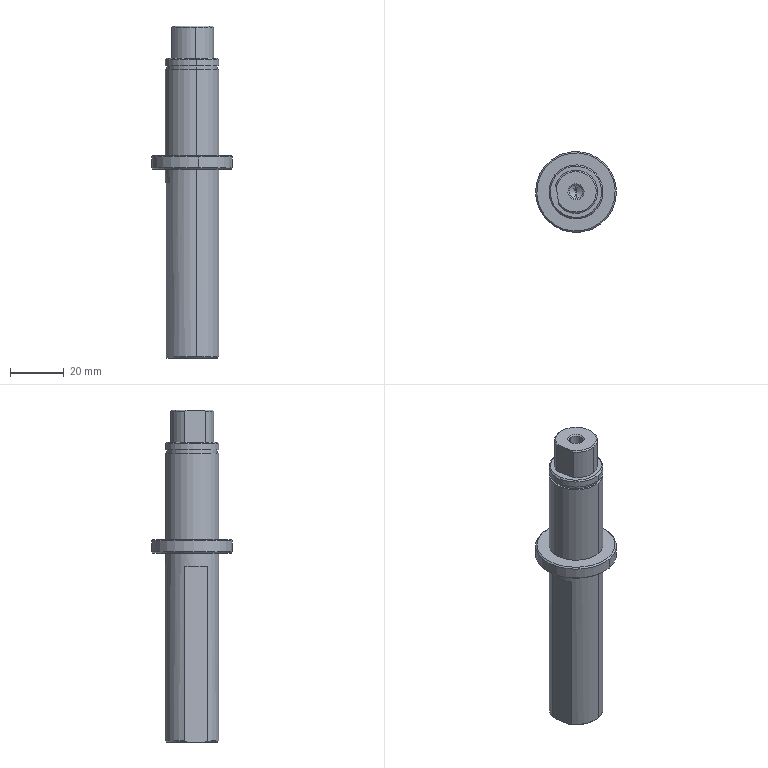Component | SolidWorks | YX-04-106GluePaperFeedingRotatingAxis-1 | 1 solid | 47 faces | box 30 x 30 x 123 mm | volume 37466 mm3 | cone 20 | cylinder 17 | plane 10 | commonest cylinder face diameters 20 x6 16 x3 5 x2 6.8 x2 18.6 x2 30 x2 | material 45#Steel
build123d program:
from build123d import *

# Parameters (mm, degrees)
SKETCH2_R                      = 10
BOSS_EXTRUDE1_DEPTH            = 70
CUT_EXTRUDE1_START             = -65
CUT_EXTRUDE1_DEPTH             = 65
BOSS_EXTRUDE2_DEPTH            = 12
F_6_8_6_8_DIAMETER_HOLE1_D     = 6.8
F_6_8_6_8_DIAMETER_HOLE1_DEPTH = 25
F_6_8_6_8_DIAMETER_HOLE1_TIP   = 2.043
F_5_0_5_DIAMETER_HOLE1_D       = 5
F_5_0_5_DIAMETER_HOLE1_DEPTH   = 15
F_5_0_5_DIAMETER_HOLE1_TIP     = 1.502
CHAMFER1_SIZE                  = 0.5
CHAMFER2_SIZE                  = 0.6


with BuildPart() as part:
    # Sketch1 → Revolve1 (revolve)
    with BuildSketch(Plane.XY, mode=Mode.PRIVATE) as revolve1_sk:
        Polygon((0, 10), (0, 0), (41, 0), (41, 15), (36, 15), (36, 10), (4, 10), (4, 9.3), (2.8, 9.3), (2.8, 10), align=None)
    revolve(revolve1_sk.sketch.rotate(Axis((0, 0, 0), (1, 0, 0)), 270), axis=Axis((0, 0, 0), (1, 0, 0)))

    # Sketch2 → Boss-Extrude1 (add)
    with BuildSketch(Plane(origin=(41, 0, 0), x_dir=(0, 0, -1), z_dir=(1, 0, 0))):
        Circle(SKETCH2_R)
    extrude(amount=BOSS_EXTRUDE1_DEPTH)

    # Sketch3 → Cut-Extrude1 (cut)
    with BuildSketch(Plane(origin=(111, 0, 0), x_dir=(0, 0, -1), z_dir=(1, 0, 0)).offset(CUT_EXTRUDE1_START)):
        with BuildLine():
            Line((-4.359, 9), (4.359, 9))
            ThreePointArc((4.359, 9), (0, 10), (-4.359, 9))
        make_face()
    extrude(amount=CUT_EXTRUDE1_DEPTH, mode=Mode.SUBTRACT)

    # Sketch4 → Boss-Extrude2 (add)
    with BuildSketch(Plane.ZY):
        with BuildLine():
            Line((-3.873, 7), (3.873, 7))
            ThreePointArc((3.873, 7), (0, -8), (-3.873, 7))
        make_face()
    extrude(amount=BOSS_EXTRUDE2_DEPTH)

    # 6.8 _6.8_ Diameter Hole1
    with Locations(Plane(origin=(111, 0, 0), x_dir=(0, 0, -1), z_dir=(1, 0, 0))):
        with Locations((0, 0)):
            Hole(F_6_8_6_8_DIAMETER_HOLE1_D / 2, depth=F_6_8_6_8_DIAMETER_HOLE1_DEPTH)
            with Locations((0, 0, -(F_6_8_6_8_DIAMETER_HOLE1_DEPTH + F_6_8_6_8_DIAMETER_HOLE1_TIP / 2))):  # 118° drill point
                Cone(0, F_6_8_6_8_DIAMETER_HOLE1_D / 2, F_6_8_6_8_DIAMETER_HOLE1_TIP, mode=Mode.SUBTRACT)

    # 5.0 _5_ Diameter Hole1
    with Locations(Plane.ZY.offset(12)):
        with Locations((0, 0)):
            Hole(F_5_0_5_DIAMETER_HOLE1_D / 2, depth=F_5_0_5_DIAMETER_HOLE1_DEPTH)
            with Locations((0, 0, -(F_5_0_5_DIAMETER_HOLE1_DEPTH + F_5_0_5_DIAMETER_HOLE1_TIP / 2))):  # 118° drill point
                Cone(0, F_5_0_5_DIAMETER_HOLE1_D / 2, F_5_0_5_DIAMETER_HOLE1_TIP, mode=Mode.SUBTRACT)

    # Chamfer1
    chamfer1_edges = [part.edges().sort_by_distance(p)[0] for p in [
        (0, 0, 10),
        (111, -8.473, 5.311),
        (-12, -8, 0),
        (-12, 0, 2.5),
        (36, 0, 15),
        (41, 0, 15),
    ]]
    chamfer(chamfer1_edges, length=CHAMFER1_SIZE)

    # Chamfer2
    chamfer2_edges = [part.edges().sort_by_distance(p)[0] for p in [
        (111, 0, -3.4),
    ]]
    chamfer(chamfer2_edges, length=CHAMFER2_SIZE)


solid = part.part

# Placed as in the assembly
solid = solid.moved(Location((-103.397, 6.262, 223), (-90, -9.843, 90)))